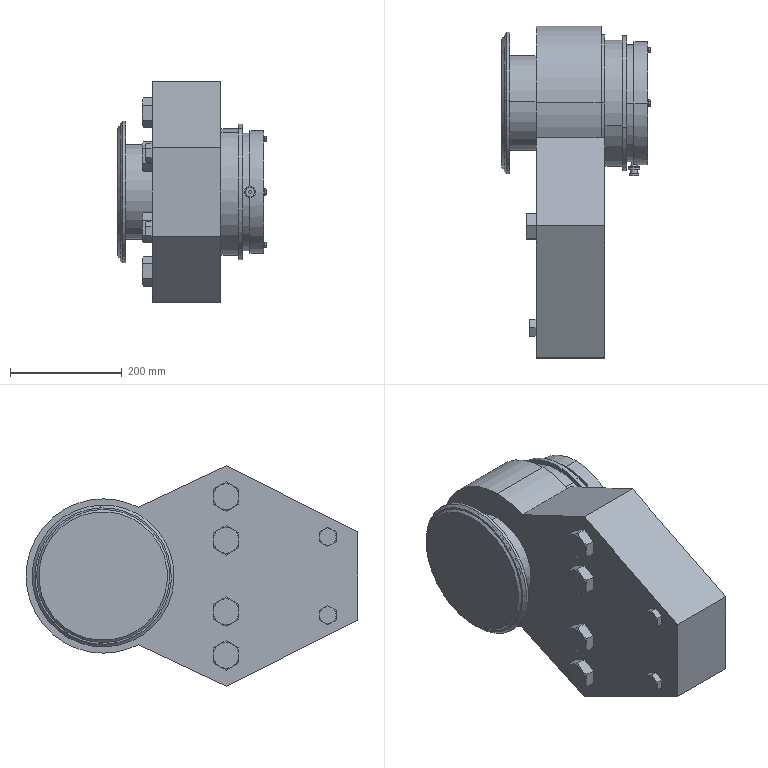Assembly | SolidWorks | mm | 24 component files | 25 solids | 523 faces | box 265.5 x 594 x 395 mm | volume 22578049 mm3 | cylinder 209 | plane 167 | cone 137 | torus 10 | commonest cylinder face diameters 34 x22 100 x22 30 x20 6 x18 5 x17 20 x12 116 x12 170 x10
Bill of materials:
AdjustingScrew | 1 |  | Thin-walled open cylindrical sleeve with a narrow, thin radial flange lip at one end.
Bracket | 1 |  | Flat thick plate with a pointed, roughly hexagonal profile on one side, merging into a circular ring lobe with a large through-bore on the other; plate carries six small through holes.
BrakeShoe | 1 |  | Thin solid circular disc with a chamfer on one edge.
CylinderEndCap | 1 |  | Axisymmetric turned part with a small central through-bore: an end collar, a smaller-diameter neck, a larger collar, and a conical taper to a truncated tip.
DiscSpring | 1 |  | Thick-walled hollow cylinder with four evenly spaced external circumferential grooves and a chamfer at one end.
EndCap | 1 |  | Stepped annular ring: a wide flange disc joined to a smaller-diameter hub, with a large central bore and small holes.
GB_T5782-2016[HexHeadBoltM20_40] | 2 |  | Short hex-head bolt-like part: a hexagonal head with chamfered outer corners, a thin round washer face or collar under the head, a small fillet where it meets the shank, and a short smooth cylindrical shank ending in a flat end.
GB_T5782-2016[HexHeadBoltM30_120] | 5 |  | Hex-head part with a stepped cylindrical shank: a chamfered hexagonal head, then a short larger-diameter cylindrical section next to the head, then a longer smaller-diameter cylindrical section ending in a flat end.
GB_T5782-2016[HexHeadBoltM6_35] | 3 |  | Long, slender hex-head bolt-like part: a chamfered hexagonal head with a thin round washer face or collar underneath, and a long plain cylindrical shank of constant diameter ending in a flat end.
Liner | 1 |  | Flanged cylindrical cup or cap: a thin-walled cylinder with a thin, edge-chamfered flange at one end, appearing closed at the flange end and open at the other.
Piston | 1 |  | Stepped cylindrical body: a smaller-diameter shaft and a larger-diameter head, with a small central through-hole and an annular recess in the head face.
PistonCylinder | 1 |  | Short, large-bore cylindrical sleeve with a stepped flange at one end, an internal groove or step in the bore, small axial holes in the end face and a small notch at the flange rim.
PistonRod | 1 |  | Bent round rod: a long straight leg with an approximately right-angle bend to a shorter leg, plus a short, thinner angled branch rod near the far end of the long leg.
SealRing1 | 1 |  | Flat annular ring with a rectangular cross-section and a moderate radial width.
SealRing2 | 1 |  | Very thin narrow ring with a small square or rectangular cross-section.
SealRing3 | 1 |  | Very thin flat annular disc (plain washer-like shape) with a single concentric circular through-hole; the hole diameter is roughly one-third of the outer diameter.
SpringSeat | 1 |  | Flat annular ring with a large concentric bore and a fairly narrow radial wall; much thicker relative to its diameter than unnamed part.
Mates:
1. coincident | Liner-1 face at (-253.5, 122.935, -3.997) dir (-1, 0, 0) | BrakeShoe-1 face at (-253.5, 95.636, 77.348) dir (1, 0, 0)
2. coincident | Liner-1 face at (-257.5, 0, 0) dir (-1, 0, 0) r 785.398 | BrakeShoe-1 face at (-253.5, 0, 0) dir (-1, 0, 0) r 785.398
3. concentric | EndCap-1 face at (-60, 0, 0) dir (1, 0, 0) r 85 | Piston-1 face at (-28.66, 0, 0) dir (1, 0, 0) r 80
4. concentric | GB_T5782-2016[HexHeadBoltM30_120]-1 face at (-22.96, 0, 0) dir (1, 0, 0) r 15 | Piston-1 face at (-28.66, 0, 0) dir (1, 0, 0) r 80
5. concentric | Piston-1 face at (-28.66, 0, 0) dir (1, 0, 0) r 80 | PistonCylinder-1 face at (-25, 0, 0) dir (1, 0, 0) r 105
6. coincident | EndCap-1 face at (-25, 0, 0) dir (-1, 0, 0) | PistonCylinder-1 face at (-25, 105, 0.000014) dir (1, 0, 0)
7. concentric | SpringSeat-1 face at (-149.5, 0, 0) dir (-1, 0, 0) r 73.5 | PistonCylinder-1 face at (-25, 0, 0) dir (1, 0, 0) r 105
8. concentric | Liner-1 face at (-257.5, 0, 0) dir (-1, 0, 0) r 85 | PistonCylinder-1 face at (-25, 0, 0) dir (1, 0, 0) r 105
9. concentric | Liner-1 face at (-257.5, 0, 0) dir (-1, 0, 0) r 85 | AdjustingScrew-1 face at (-126, 0, 0) dir (-1, 0, 0) r 113
10. coincident | EndCap-1 plane at (0, 0, 0) dir (0, 0, -1) | assembly plane at (0, 0, 0) dir (0, 0, 1)
11. coincident | EndCap-1 plane at (0, 0, 0) dir (0, 1, 0) | assembly plane at (0, 0, 0) dir (0, 1, 0)
12. coincident | EndCap-1 plane at (0, 0, 0) dir (-1, 0, 0) | assembly plane at (0, 0, 0) dir (1, 0, 0)
13. concentric | PistonCylinder-1 face at (-25, 0, 0) dir (1, 0, 0) r 105 | SealRing1-1 face at (-130.5, 0, 0) dir (-1, 0, 0) r 58
14. coincident | PistonCylinder-1 face at (-130.5, 50, 0.000006) dir (-1, 0, 0) | SealRing1-1 face at (-130.5, 0, 0) dir (1, 0, 0)
15. coincident | SpringSeat-1 face at (-138, 29.938, -59.939) dir (1, 0, 0) | SealRing1-1 face at (-138, 0, 0) dir (-1, 0, 0)
16. concentric | PistonCylinder-1 face at (-25, 0, 0) dir (1, 0, 0) r 105 | SealRing2-1 face at (-60, 0, 0) dir (-1, 0, 0) r 85
17. coincident | EndCap-1 face at (-60, 0, 0) dir (-1, 0, 0) | SealRing2-1 face at (-60, 0, 0) dir (1, 0, 0)
18. coincident | GB_T5782-2016[HexHeadBoltM30_120]-1 face at (-73.66, 0, 0) dir (-1, 0, 0) | Piston-1 face at (-73.66, 1.475, -9.891) dir (1, 0, 0)
19. concentric | Piston-1 face at (-28.66, 0, 0) dir (1, 0, 0) r 80 | SealRing3-1 face at (-41.66, 0, 0) dir (-1, 0, 0) r 48.5
20. coincident | Piston-1 face at (-43.66, 7.377, -49.453) dir (1, 0, 0) | SealRing3-1 face at (-43.66, 0, 0) dir (-1, 0, 0)
21. coincident | AdjustingScrew-1 face at (-126, 105.697, 39.964) dir (-1, 0, 0) | PistonCylinder-1 face at (-126, 110.5, 0.000014) dir (1, 0, 0)
22. coincident | Bracket-1 plane at (-199.5, 0, 0) dir (0, 0, 1) | assembly plane at (0, 0, 0) dir (0, 0, 1)
23. coincident | Liner-1 face at (-149.5, 74.96, -2.437) dir (1, 0, 0) | SpringSeat-1 face at (-149.5, 31.502, -63.07) dir (-1, 0, 0)
24. coincident | Bracket-1 plane at (-199.5, 0, 0) dir (0, -1, 0) | assembly plane at (0, 0, 0) dir (0, 1, 0)
25. distance | Bracket-1 face at (-199.5, 0, 0) dir (-1, 0, 0) | Liner-1 face at (-149.5, 74.96, -2.437) dir (1, 0, 0)
26. concentric | AdjustingScrew-1 face at (-126, 0, 0) dir (-1, 0, 0) r 113 | DiscSpring-1 face at (-157.396, 0, 0) dir (1, 0, 0) r 70
27. coincident | SpringSeat-1 face at (-147, 0, 0) dir (1, 0, 0) r 1413.717 | DiscSpring-1 face at (-146.129, 0, 0) dir (1, 0, 0) r 1413.717
28. concentric | Bracket-1 face at (-199.5, -402, 70) dir (-1, 0, 0) r 10 | GB_T5782-2016[HexHeadBoltM20_40]-1 face at (-212, -402, 70) dir (-1, 0, 0) r 10
29. coincident | Bracket-1 face at (-199.5, 0, 0) dir (-1, 0, 0) | GB_T5782-2016[HexHeadBoltM20_40]-1 face at (-199.5, -387, 61.34) dir (1, 0, 0)
30. concentric | Bracket-1 face at (-199.5, -220, -64) dir (-1, 0, 0) r 15 | GB_T5782-2016[HexHeadBoltM30_120]-2 face at (-218.2, -220, -64) dir (-1, 0, 0) r 15
31. coincident | Bracket-1 face at (-199.5, 0, 0) dir (-1, 0, 0) | GB_T5782-2016[HexHeadBoltM30_120]-2 face at (-199.5, -197, -77.279) dir (1, 0, 0)
32. concentric | Bracket-1 face at (-199.5, -220, 64) dir (-1, 0, 0) r 15 | GB_T5782-2016[HexHeadBoltM30_120]-4 face at (-218.2, -220, 64) dir (-1, 0, 0) r 15
33. coincident | GB_T5782-2016[HexHeadBoltM30_120]-2 face at (-218.2, -197, -77.279) dir (-1, 0, 0) | GB_T5782-2016[HexHeadBoltM30_120]-4 face at (-218.2, -197, 50.721) dir (-1, 0, 0)
34. coincident | GB_T5782-2016[HexHeadBoltM20_40]-1 face at (-212, -387, 61.34) dir (-1, 0, 0) | GB_T5782-2016[HexHeadBoltM20_40]-2 face at (-212, -387, -78.66) dir (-1, 0, 0)
35. concentric | Bracket-1 face at (-199.5, -402, -70) dir (-1, 0, 0) r 10 | GB_T5782-2016[HexHeadBoltM20_40]-2 face at (-212, -402, -70) dir (-1, 0, 0) r 10
36. coincident | GB_T5782-2016[HexHeadBoltM30_120]-2 face at (-199.5, -197, -77.279) dir (0, 1, 0) | GB_T5782-2016[HexHeadBoltM30_120]-4 face at (-199.5, -197, 50.721) dir (0, 1, 0)
37. coincident | GB_T5782-2016[HexHeadBoltM20_40]-1 face at (-199.5, -387, 61.34) dir (0, 1, 0) | GB_T5782-2016[HexHeadBoltM20_40]-2 face at (-199.5, -387, -78.66) dir (0, 1, 0)
38. concentric | Bracket-1 face at (-199.5, -220, -142) dir (-1, 0, 0) r 15 | GB_T5782-2016[HexHeadBoltM30_120]-6 face at (-218.2, -220, -142) dir (-1, 0, 0) r 15
39. concentric | Bracket-1 face at (-199.5, -220, 142) dir (-1, 0, 0) r 15 | GB_T5782-2016[HexHeadBoltM30_120]-5 face at (-218.2, -220, 142) dir (-1, 0, 0) r 15
40. coincident | GB_T5782-2016[HexHeadBoltM30_120]-5 face at (-218.2, -220, 168.558) dir (-1, 0, 0) | GB_T5782-2016[HexHeadBoltM30_120]-6 face at (-218.2, -197, -128.721) dir (-1, 0, 0)
41. coincident | GB_T5782-2016[HexHeadBoltM30_120]-2 face at (-218.2, -197, -77.279) dir (-1, 0, 0) | GB_T5782-2016[HexHeadBoltM30_120]-6 face at (-218.2, -197, -128.721) dir (-1, 0, 0)
42. coincident | GB_T5782-2016[HexHeadBoltM30_120]-5 face at (-199.5, -197, 155.279) dir (0, 1, 0) | GB_T5782-2016[HexHeadBoltM30_120]-6 face at (-199.5, -197, -155.279) dir (0, 1, 0)
43. concentric | CylinderEndCap-1 face at (-25, -95, 0) dir (0, -1, 0) r 2.5 | PistonRod-1 face at (-25, -130, 0) dir (0, 1, 0) r 2.5
44. coincident | CylinderEndCap-1 face at (-17.081, -130, -3.09) dir (0, -1, 0) | PistonRod-1 face at (-25, -130, 0) dir (0, -1, 0)
45. coincident | PistonRod-1 plane at (-25, -95, 0) dir (0, 0, -1) | assembly plane at (0, 0, 0) dir (0, 0, 1)
46. coincident | EndCap-1 sketch point at (-25, -95, 0) dir (1, 0, 0) | PistonRod-1 sketch segment at (-25, -95, 0) dir (-1, 0, 0)
47. parallel | PistonRod-1 plane at (-25, -95, 0) dir (0, -1, 0) | assembly plane at (0, 0, 0) dir (0, 1, 0)
48. coincident | EndCap-1 face at (-25, 0, 0) dir (-1, 0, 0) | PistonRod-1 sketch segment at (-25, -95, 0) dir (0, -1, 0)
49. coincident | EndCap-1 face at (0, 0, 0) dir (1, 0, 0) | GB_T5782-2016[HexHeadBoltM6_35]-1 face at (0, 100, -2.887) dir (-1, 0, 0)
50. concentric | EndCap-1 face at (0, 95, 0) dir (-1, 0, 0) r 3 | GB_T5782-2016[HexHeadBoltM6_35]-1 face at (4, 95, 0) dir (1, 0, 0) r 3
51. parallel | Bracket-1 face at (-77.5, -456, 78.811) dir (0, -1, 0) | GB_T5782-2016[HexHeadBoltM6_35]-1 face at (0, 100, 2.887) dir (0, 1, 0)